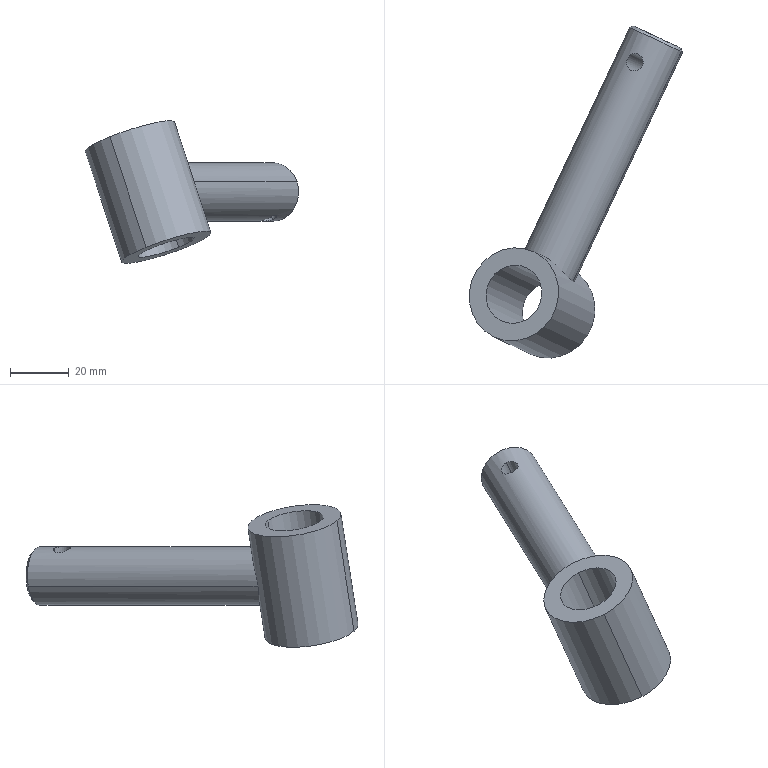Component | SolidWorks | FilmPressingSoilCoveringMechanism2Reverse-2_AttachedSoilWheelVerticalAxis2-1 | 1 solid | 13 faces | box 72.68 x 113.03 x 48.53 mm | volume 45663 mm3 | cylinder 8 | plane 3 | cone 2 | commonest cylinder face diameters 20 x4 6 x2 32 x2
build123d program:
from build123d import *

# Parameters (mm, degrees)
SKETCH1_R           = 16
BOSS_EXTRUDE1_DEPTH = 20
SKETCH2_R           = 10
BOSS_EXTRUDE2_DEPTH = 100
CHAMFER1_SIZE       = 1
SKETCH3_R           = 3
CUT_EXTRUDE1_DEPTH  = 50
SKETCH4_R           = 10
CUT_EXTRUDE2_DEPTH  = 109.885


with BuildPart() as part:
    # Sketch1 → Boss-Extrude1 (new, symmetric)
    with BuildSketch(Plane(origin=(0, 0, 0), x_dir=(1, 0, 0), z_dir=(0, 1, 0))):
        with Locations(Location((0, 0, 0), (0, 0, 270))):
            Circle(SKETCH1_R)
    extrude(amount=BOSS_EXTRUDE1_DEPTH, both=True)

    # Sketch2 → Boss-Extrude2 (add)
    with BuildSketch(Plane.XY):
        with Locations(Location((0, 0, 0), (0, 0, 180))):
            Circle(SKETCH2_R)
    extrude(amount=BOSS_EXTRUDE2_DEPTH)

    # Chamfer1
    chamfer1_edges = [part.edges().sort_by_distance(p)[0] for p in [
        (10, 0, 100),
    ]]
    chamfer(chamfer1_edges, length=CHAMFER1_SIZE)

    # Sketch3 → Cut-Extrude1 (cut, symmetric)
    with BuildSketch(Plane(origin=(0, 0, 0), x_dir=(1, 0, 0), z_dir=(0, 1, 0))):
        with Locations(Location((0, -89, 0), (0, 0, 270))):
            Circle(SKETCH3_R)
    extrude(amount=CUT_EXTRUDE1_DEPTH, both=True, mode=Mode.SUBTRACT)

    # Sketch4 → Cut-Extrude2 (cut, through all)
    with BuildSketch(Plane(origin=(0, 20, 0), x_dir=(1, 0, 0), z_dir=(0, 1, 0))):
        with Locations(Location((0, 0, 0), (0, 0, 270))):
            Circle(SKETCH4_R)
    extrude(amount=-CUT_EXTRUDE2_DEPTH, mode=Mode.SUBTRACT)


solid = part.part

# Placed as in the assembly
solid = solid.moved(Location((-1911.671, -307.604, 2567.971), (-90, 25.252, -20)))
STEP:
#1=COLOUR_RGB('',0.7922,0.8196,0.9333);
#2=FILL_AREA_STYLE_COLOUR('',#1);
#3=FILL_AREA_STYLE('',(#2));
#4=SURFACE_STYLE_FILL_AREA(#3);
#5=SURFACE_SIDE_STYLE('',(#4));
#6=SURFACE_STYLE_USAGE(.BOTH.,#5);
#7=PRESENTATION_STYLE_ASSIGNMENT((#6));
#8=CARTESIAN_POINT('',(-75.674,-12.352,101.841));
#9=VERTEX_POINT('',#8);
#10=CARTESIAN_POINT('',(-75.338,-11.639,101.841));
#11=VERTEX_POINT('',#10);
#12=CARTESIAN_POINT('',(-75.506,-11.995,101.841));
#13=DIRECTION('',(0.3093,-0.1459,-0.9397));
#14=DIRECTION('',(0.4266,0.9044,0.));
#15=AXIS2_PLACEMENT_3D('',#12,#13,#14);
#16=CIRCLE('',#15,0.3937);
#17=EDGE_CURVE('',#9,#11,#16,.T.);
#18=ORIENTED_EDGE('',*,*,#17,.F.);
#19=CARTESIAN_POINT('',(-75.187,-12.581,100.361));
#20=VERTEX_POINT('',#19);
#21=CARTESIAN_POINT('',(-75.674,-12.352,101.841));
#22=DIRECTION('',(0.3093,-0.1459,-0.9397));
#23=VECTOR('',#22,39.37);
#24=LINE('',#21,#23);
#25=EDGE_CURVE('',#9,#20,#24,.T.);
#26=ORIENTED_EDGE('',*,*,#25,.T.);
#27=CARTESIAN_POINT('',(-74.851,-11.869,100.361));
#28=VERTEX_POINT('',#27);
#29=CARTESIAN_POINT('',(-75.019,-12.225,100.361));
#30=DIRECTION('',(0.3093,-0.1459,-0.9397));
#31=DIRECTION('',(0.4266,0.9044,0.));
#32=AXIS2_PLACEMENT_3D('',#29,#30,#31);
#33=CIRCLE('',#32,0.3937);
#34=EDGE_CURVE('',#20,#28,#33,.T.);
#35=ORIENTED_EDGE('',*,*,#34,.T.);
#36=CARTESIAN_POINT('',(-75.338,-11.639,101.841));
#37=DIRECTION('',(0.3093,-0.1459,-0.9397));
#38=VECTOR('',#37,39.37);
#39=LINE('',#36,#38);
#40=EDGE_CURVE('',#11,#28,#39,.T.);
#41=ORIENTED_EDGE('',*,*,#40,.F.);
#42=EDGE_LOOP('',(#18,#26,#35,#41));
#43=FACE_OUTER_BOUND('',#42,.T.);
#44=CARTESIAN_POINT('',(-75.506,-11.995,101.841));
#45=DIRECTION('',(0.3093,-0.1459,-0.9397));
#46=DIRECTION('',(0.4266,0.9044,0.));
#47=AXIS2_PLACEMENT_3D('',#44,#45,#46);
#48=CYLINDRICAL_SURFACE('',#47,0.3937);
#49=ADVANCED_FACE('',(#43),#48,.F.);
#50=CARTESIAN_POINT('',(-73.94,-8.991,101.471));
#51=VERTEX_POINT('',#50);
#52=CARTESIAN_POINT('',(-73.839,-8.777,101.471));
#53=VERTEX_POINT('',#52);
#54=CARTESIAN_POINT('',(-73.94,-8.991,101.471));
#55=CARTESIAN_POINT('',(-73.947,-8.988,101.469));
#56=CARTESIAN_POINT('',(-73.953,-8.984,101.466));
#57=CARTESIAN_POINT('',(-73.964,-8.975,101.46));
#58=CARTESIAN_POINT('',(-73.969,-8.97,101.456));
#59=CARTESIAN_POINT('',(-73.978,-8.959,101.45));
#60=CARTESIAN_POINT('',(-73.982,-8.953,101.447));
#61=CARTESIAN_POINT('',(-73.989,-8.941,101.44));
#62=CARTESIAN_POINT('',(-73.992,-8.934,101.437));
#63=CARTESIAN_POINT('',(-73.995,-8.92,101.431));
#64=CARTESIAN_POINT('',(-73.997,-8.913,101.428));
#65=CARTESIAN_POINT('',(-73.998,-8.898,101.423));
#66=CARTESIAN_POINT('',(-73.998,-8.891,101.421));
#67=CARTESIAN_POINT('',(-73.996,-8.876,101.418));
#68=CARTESIAN_POINT('',(-73.995,-8.868,101.416));
#69=CARTESIAN_POINT('',(-73.99,-8.854,101.414));
#70=CARTESIAN_POINT('',(-73.988,-8.846,101.414));
#71=CARTESIAN_POINT('',(-73.981,-8.832,101.414));
#72=CARTESIAN_POINT('',(-73.977,-8.825,101.414));
#73=CARTESIAN_POINT('',(-73.968,-8.813,101.416));
#74=CARTESIAN_POINT('',(-73.964,-8.807,101.418));
#75=CARTESIAN_POINT('',(-73.948,-8.791,101.423));
#76=CARTESIAN_POINT('',(-73.935,-8.782,101.428));
#77=CARTESIAN_POINT('',(-73.916,-8.773,101.437));
#78=CARTESIAN_POINT('',(-73.909,-8.771,101.44));
#79=CARTESIAN_POINT('',(-73.895,-8.768,101.447));
#80=CARTESIAN_POINT('',(-73.888,-8.767,101.45));
#81=CARTESIAN_POINT('',(-73.874,-8.767,101.456));
#82=CARTESIAN_POINT('',(-73.867,-8.768,101.46));
#83=CARTESIAN_POINT('',(-73.853,-8.772,101.466));
#84=CARTESIAN_POINT('',(-73.846,-8.774,101.469));
#85=CARTESIAN_POINT('',(-73.839,-8.777,101.471));
#86=B_SPLINE_CURVE_WITH_KNOTS('',3,(#54,#55,#56,#57,#58,#59,#60,#61,#62,#63,#64,#65,#66,#67,#68,#69,#70,#71,#72,#73,#74,#75,#76,#77,#78,#79,#80,#81,#82,#83,#84,#85),.UNSPECIFIED.,.F.,.F.,(4,2,2,2,2,2,2,2,2,2,2,2,2,2,2,4),(0.009434,0.01002,0.01061,0.0112,0.01179,0.01238,0.01297,0.01356,0.01415,0.01474,0.01533,0.01651,0.0171,0.01769,0.01828,0.01887),.UNSPECIFIED.);
#87=EDGE_CURVE('',#51,#53,#86,.T.);
#88=ORIENTED_EDGE('',*,*,#87,.F.);
#89=CARTESIAN_POINT('',(-73.696,-9.106,100.731));
#90=VERTEX_POINT('',#89);
#91=CARTESIAN_POINT('',(-74.427,-8.761,102.951));
#92=DIRECTION('',(0.3093,-0.1459,-0.9397));
#93=VECTOR('',#92,39.37);
#94=LINE('',#91,#93);
#95=EDGE_CURVE('',#51,#90,#94,.T.);
#96=ORIENTED_EDGE('',*,*,#95,.T.);
#97=CARTESIAN_POINT('',(-73.596,-8.892,100.731));
#98=VERTEX_POINT('',#97);
#99=CARTESIAN_POINT('',(-73.596,-8.892,100.731));
#100=CARTESIAN_POINT('',(-73.602,-8.889,100.729));
#101=CARTESIAN_POINT('',(-73.609,-8.886,100.726));
#102=CARTESIAN_POINT('',(-73.624,-8.883,100.722));
#103=CARTESIAN_POINT('',(-73.631,-8.882,100.72));
#104=CARTESIAN_POINT('',(-73.647,-8.881,100.717));
#105=CARTESIAN_POINT('',(-73.654,-8.882,100.715));
#106=CARTESIAN_POINT('',(-73.669,-8.884,100.713));
#107=CARTESIAN_POINT('',(-73.677,-8.886,100.712));
#108=CARTESIAN_POINT('',(-73.699,-8.894,100.71));
#109=CARTESIAN_POINT('',(-73.713,-8.902,100.709));
#110=CARTESIAN_POINT('',(-73.73,-8.917,100.708));
#111=CARTESIAN_POINT('',(-73.735,-8.923,100.708));
#112=CARTESIAN_POINT('',(-73.745,-8.935,100.708));
#113=CARTESIAN_POINT('',(-73.749,-8.942,100.708));
#114=CARTESIAN_POINT('',(-73.755,-8.956,100.708));
#115=CARTESIAN_POINT('',(-73.758,-8.963,100.708));
#116=CARTESIAN_POINT('',(-73.762,-8.978,100.708));
#117=CARTESIAN_POINT('',(-73.763,-8.986,100.708));
#118=CARTESIAN_POINT('',(-73.763,-9.002,100.709));
#119=CARTESIAN_POINT('',(-73.763,-9.009,100.709));
#120=CARTESIAN_POINT('',(-73.76,-9.025,100.71));
#121=CARTESIAN_POINT('',(-73.758,-9.032,100.71));
#122=CARTESIAN_POINT('',(-73.753,-9.047,100.712));
#123=CARTESIAN_POINT('',(-73.749,-9.054,100.713));
#124=CARTESIAN_POINT('',(-73.742,-9.067,100.715));
#125=CARTESIAN_POINT('',(-73.737,-9.073,100.717));
#126=CARTESIAN_POINT('',(-73.727,-9.084,100.72));
#127=CARTESIAN_POINT('',(-73.721,-9.09,100.722));
#128=CARTESIAN_POINT('',(-73.709,-9.099,100.726));
#129=CARTESIAN_POINT('',(-73.703,-9.102,100.729));
#130=CARTESIAN_POINT('',(-73.696,-9.106,100.731));
#131=B_SPLINE_CURVE_WITH_KNOTS('',3,(#99,#100,#101,#102,#103,#104,#105,#106,#107,#108,#109,#110,#111,#112,#113,#114,#115,#116,#117,#118,#119,#120,#121,#122,#123,#124,#125,#126,#127,#128,#129,#130),.UNSPECIFIED.,.F.,.F.,(4,2,2,2,2,2,2,2,2,2,2,2,2,2,2,4),(0.,0.0005896,0.001179,0.001769,0.002359,0.003538,0.004127,0.004717,0.005307,0.005896,0.006486,0.007076,0.007665,0.008255,0.008844,0.009434),.UNSPECIFIED.);
#132=EDGE_CURVE('',#98,#90,#131,.T.);
#133=ORIENTED_EDGE('',*,*,#132,.F.);
#134=CARTESIAN_POINT('',(-74.326,-8.547,102.951));
#135=DIRECTION('',(0.3093,-0.1459,-0.9397));
#136=VECTOR('',#135,39.37);
#137=LINE('',#134,#136);
#138=EDGE_CURVE('',#53,#98,#137,.T.);
#139=ORIENTED_EDGE('',*,*,#138,.F.);
#140=EDGE_LOOP('',(#88,#96,#133,#139));
#141=FACE_OUTER_BOUND('',#140,.T.);
#142=CARTESIAN_POINT('',(-74.377,-8.654,102.951));
#143=DIRECTION('',(0.3093,-0.1459,-0.9397));
#144=DIRECTION('',(0.4266,0.9044,0.));
#145=AXIS2_PLACEMENT_3D('',#142,#143,#144);
#146=CYLINDRICAL_SURFACE('',#145,0.1181);
#147=ADVANCED_FACE('',(#141),#146,.F.);
#148=CARTESIAN_POINT('',(-73.282,-8.692,101.222));
#149=VERTEX_POINT('',#148);
#150=CARTESIAN_POINT('',(-73.884,-8.408,100.98));
#151=VERTEX_POINT('',#150);
#152=CARTESIAN_POINT('',(-73.583,-8.55,101.101));
#153=DIRECTION('',(0.4266,0.9044,0.));
#154=DIRECTION('',(0.8499,-0.4009,0.342));
#155=AXIS2_PLACEMENT_3D('',#152,#153,#154);
#156=CIRCLE('',#155,0.3543);
#157=EDGE_CURVE('',#149,#151,#156,.T.);
#158=ORIENTED_EDGE('',*,*,#157,.F.);
#159=CARTESIAN_POINT('',(-73.265,-8.743,101.236));
#160=VERTEX_POINT('',#159);
#161=CARTESIAN_POINT('',(-73.282,-8.692,101.222));
#162=DIRECTION('',(0.2993,-0.923,0.2418));
#163=VECTOR('',#162,39.37);
#164=LINE('',#161,#163);
#165=EDGE_CURVE('',#149,#160,#164,.T.);
#166=ORIENTED_EDGE('',*,*,#165,.T.);
#167=CARTESIAN_POINT('',(-73.935,-8.427,100.967));
#168=VERTEX_POINT('',#167);
#169=CARTESIAN_POINT('',(-73.6,-8.585,101.101));
#170=DIRECTION('',(-0.4266,-0.9044,-0.));
#171=DIRECTION('',(0.8499,-0.4009,0.342));
#172=AXIS2_PLACEMENT_3D('',#169,#170,#171);
#173=CIRCLE('',#172,0.3937);
#174=EDGE_CURVE('',#168,#160,#173,.T.);
#175=ORIENTED_EDGE('',*,*,#174,.F.);
#176=CARTESIAN_POINT('',(-73.884,-8.408,100.98));
#177=DIRECTION('',(-0.9026,-0.3561,-0.2418));
#178=VECTOR('',#177,39.37);
#179=LINE('',#176,#178);
#180=EDGE_CURVE('',#151,#168,#179,.T.);
#181=ORIENTED_EDGE('',*,*,#180,.F.);
#182=EDGE_LOOP('',(#158,#166,#175,#181));
#183=FACE_OUTER_BOUND('',#182,.T.);
#184=CARTESIAN_POINT('',(-73.583,-8.55,101.101));
#185=DIRECTION('',(-0.4266,-0.9044,-0.));
#186=DIRECTION('',(-0.8499,0.4009,-0.342));
#187=AXIS2_PLACEMENT_3D('',#184,#185,#186);
#188=CONICAL_SURFACE('',#187,0.3543,0.7854);
#189=ADVANCED_FACE('',(#183),#188,.T.);
#190=ORIENTED_EDGE('',*,*,#132,.T.);
#191=CARTESIAN_POINT('',(-73.696,-9.106,100.731));
#192=CARTESIAN_POINT('',(-73.69,-9.109,100.734));
#193=CARTESIAN_POINT('',(-73.683,-9.111,100.737));
#194=CARTESIAN_POINT('',(-73.669,-9.114,100.743));
#195=CARTESIAN_POINT('',(-73.662,-9.115,100.746));
#196=CARTESIAN_POINT('',(-73.648,-9.115,100.752));
#197=CARTESIAN_POINT('',(-73.641,-9.114,100.756));
#198=CARTESIAN_POINT('',(-73.627,-9.112,100.762));
#199=CARTESIAN_POINT('',(-73.62,-9.109,100.765));
#200=CARTESIAN_POINT('',(-73.607,-9.104,100.771));
#201=CARTESIAN_POINT('',(-73.601,-9.1,100.774));
#202=CARTESIAN_POINT('',(-73.589,-9.091,100.779));
#203=CARTESIAN_POINT('',(-73.583,-9.087,100.781));
#204=CARTESIAN_POINT('',(-73.572,-9.076,100.785));
#205=CARTESIAN_POINT('',(-73.567,-9.07,100.786));
#206=CARTESIAN_POINT('',(-73.559,-9.057,100.788));
#207=CARTESIAN_POINT('',(-73.555,-9.05,100.789));
#208=CARTESIAN_POINT('',(-73.548,-9.036,100.789));
#209=CARTESIAN_POINT('',(-73.545,-9.029,100.788));
#210=CARTESIAN_POINT('',(-73.541,-9.014,100.786));
#211=CARTESIAN_POINT('',(-73.54,-9.007,100.785));
#212=CARTESIAN_POINT('',(-73.537,-8.984,100.779));
#213=CARTESIAN_POINT('',(-73.538,-8.969,100.774));
#214=CARTESIAN_POINT('',(-73.544,-8.949,100.765));
#215=CARTESIAN_POINT('',(-73.547,-8.942,100.762));
#216=CARTESIAN_POINT('',(-73.553,-8.929,100.756));
#217=CARTESIAN_POINT('',(-73.557,-8.923,100.752));
#218=CARTESIAN_POINT('',(-73.566,-8.913,100.746));
#219=CARTESIAN_POINT('',(-73.572,-8.908,100.743));
#220=CARTESIAN_POINT('',(-73.583,-8.899,100.737));
#221=CARTESIAN_POINT('',(-73.589,-8.895,100.734));
#222=CARTESIAN_POINT('',(-73.596,-8.892,100.731));
#223=B_SPLINE_CURVE_WITH_KNOTS('',3,(#191,#192,#193,#194,#195,#196,#197,#198,#199,#200,#201,#202,#203,#204,#205,#206,#207,#208,#209,#210,#211,#212,#213,#214,#215,#216,#217,#218,#219,#220,#221,#222),.UNSPECIFIED.,.F.,.F.,(4,2,2,2,2,2,2,2,2,2,2,2,2,2,2,4),(0.009434,0.01002,0.01061,0.0112,0.01179,0.01238,0.01297,0.01356,0.01415,0.01474,0.01533,0.01651,0.0171,0.01769,0.01828,0.01887),.UNSPECIFIED.);
#224=EDGE_CURVE('',#90,#98,#223,.T.);
#225=ORIENTED_EDGE('',*,*,#224,.T.);
#226=EDGE_LOOP('',(#190,#225));
#227=FACE_BOUND('',#226,.T.);
#228=ORIENTED_EDGE('',*,*,#174,.T.);
#229=CARTESIAN_POINT('',(-74.718,-11.823,101.236));
#230=VERTEX_POINT('',#229);
#231=CARTESIAN_POINT('',(-73.249,-8.707,101.236));
#232=DIRECTION('',(-0.4266,-0.9044,-0.));
#233=VECTOR('',#232,39.37);
#234=LINE('',#231,#233);
#235=EDGE_CURVE('',#160,#230,#234,.T.);
#236=ORIENTED_EDGE('',*,*,#235,.T.);
#237=CARTESIAN_POINT('',(-74.872,-11.598,100.731));
#238=VERTEX_POINT('',#237);
#239=CARTESIAN_POINT('',(-74.718,-11.823,101.236));
#240=CARTESIAN_POINT('',(-74.71,-11.827,101.211));
#241=CARTESIAN_POINT('',(-74.703,-11.828,101.185));
#242=CARTESIAN_POINT('',(-74.695,-11.825,101.146));
#243=CARTESIAN_POINT('',(-74.693,-11.823,101.133));
#244=CARTESIAN_POINT('',(-74.69,-11.819,101.107));
#245=CARTESIAN_POINT('',(-74.688,-11.816,101.094));
#246=CARTESIAN_POINT('',(-74.685,-11.805,101.056));
#247=CARTESIAN_POINT('',(-74.685,-11.796,101.031));
#248=CARTESIAN_POINT('',(-74.689,-11.776,100.982));
#249=CARTESIAN_POINT('',(-74.693,-11.764,100.958));
#250=CARTESIAN_POINT('',(-74.702,-11.746,100.924));
#251=CARTESIAN_POINT('',(-74.705,-11.739,100.913));
#252=CARTESIAN_POINT('',(-74.713,-11.726,100.891));
#253=CARTESIAN_POINT('',(-74.718,-11.719,100.88));
#254=CARTESIAN_POINT('',(-74.733,-11.699,100.85));
#255=CARTESIAN_POINT('',(-74.745,-11.686,100.831));
#256=CARTESIAN_POINT('',(-74.774,-11.659,100.795));
#257=CARTESIAN_POINT('',(-74.791,-11.645,100.779));
#258=CARTESIAN_POINT('',(-74.819,-11.627,100.759));
#259=CARTESIAN_POINT('',(-74.829,-11.621,100.753));
#260=CARTESIAN_POINT('',(-74.85,-11.609,100.741));
#261=CARTESIAN_POINT('',(-74.861,-11.603,100.736));
#262=CARTESIAN_POINT('',(-74.872,-11.598,100.731));
#263=B_SPLINE_CURVE_WITH_KNOTS('',3,(#239,#240,#241,#242,#243,#244,#245,#246,#247,#248,#249,#250,#251,#252,#253,#254,#255,#256,#257,#258,#259,#260,#261,#262),.UNSPECIFIED.,.F.,.F.,(4,2,2,2,2,2,2,2,2,2,2,4),(0.03215,0.03416,0.03516,0.03616,0.03817,0.04017,0.04118,0.04218,0.04419,0.04619,0.0472,0.0482),.UNSPECIFIED.);
#264=EDGE_CURVE('',#230,#238,#263,.T.);
#265=ORIENTED_EDGE('',*,*,#264,.T.);
#266=CARTESIAN_POINT('',(-75.387,-11.508,100.967));
#267=VERTEX_POINT('',#266);
#268=CARTESIAN_POINT('',(-74.872,-11.598,100.731));
#269=CARTESIAN_POINT('',(-74.895,-11.587,100.722));
#270=CARTESIAN_POINT('',(-74.919,-11.578,100.716));
#271=CARTESIAN_POINT('',(-74.956,-11.566,100.71));
#272=CARTESIAN_POINT('',(-74.969,-11.562,100.709));
#273=CARTESIAN_POINT('',(-74.994,-11.555,100.707));
#274=CARTESIAN_POINT('',(-75.007,-11.552,100.707));
#275=CARTESIAN_POINT('',(-75.033,-11.546,100.709));
#276=CARTESIAN_POINT('',(-75.046,-11.544,100.71));
#277=CARTESIAN_POINT('',(-75.072,-11.539,100.714));
#278=CARTESIAN_POINT('',(-75.085,-11.538,100.716));
#279=CARTESIAN_POINT('',(-75.123,-11.532,100.726));
#280=CARTESIAN_POINT('',(-75.148,-11.53,100.734));
#281=CARTESIAN_POINT('',(-75.185,-11.527,100.75));
#282=CARTESIAN_POINT('',(-75.197,-11.527,100.756));
#283=CARTESIAN_POINT('',(-75.22,-11.525,100.769));
#284=CARTESIAN_POINT('',(-75.231,-11.525,100.776));
#285=CARTESIAN_POINT('',(-75.264,-11.523,100.798));
#286=CARTESIAN_POINT('',(-75.285,-11.523,100.814));
#287=CARTESIAN_POINT('',(-75.313,-11.521,100.843));
#288=CARTESIAN_POINT('',(-75.322,-11.52,100.852));
#289=CARTESIAN_POINT('',(-75.339,-11.519,100.873));
#290=CARTESIAN_POINT('',(-75.346,-11.518,100.884));
#291=CARTESIAN_POINT('',(-75.36,-11.516,100.906));
#292=CARTESIAN_POINT('',(-75.367,-11.515,100.918));
#293=CARTESIAN_POINT('',(-75.378,-11.511,100.942));
#294=CARTESIAN_POINT('',(-75.383,-11.51,100.954));
#295=CARTESIAN_POINT('',(-75.387,-11.508,100.967));
#296=B_SPLINE_CURVE_WITH_KNOTS('',3,(#268,#269,#270,#271,#272,#273,#274,#275,#276,#277,#278,#279,#280,#281,#282,#283,#284,#285,#286,#287,#288,#289,#290,#291,#292,#293,#294,#295),.UNSPECIFIED.,.F.,.F.,(4,2,2,2,2,2,2,2,2,2,2,2,2,4),(0.0482,0.0502,0.0512,0.0522,0.0532,0.0542,0.05621,0.05721,0.05821,0.06021,0.06121,0.06221,0.06321,0.06421),.UNSPECIFIED.);
#297=EDGE_CURVE('',#238,#267,#296,.T.);
#298=ORIENTED_EDGE('',*,*,#297,.T.);
#299=CARTESIAN_POINT('',(-73.918,-8.392,100.967));
#300=DIRECTION('',(-0.4266,-0.9044,-0.));
#301=VECTOR('',#300,39.37);
#302=LINE('',#299,#301);
#303=EDGE_CURVE('',#168,#267,#302,.T.);
#304=ORIENTED_EDGE('',*,*,#303,.F.);
#305=EDGE_LOOP('',(#228,#236,#265,#298,#304));
#306=FACE_OUTER_BOUND('',#305,.T.);
#307=CARTESIAN_POINT('',(-73.583,-8.55,101.101));
#308=DIRECTION('',(-0.4266,-0.9044,-0.));
#309=DIRECTION('',(-0.8499,0.4009,-0.342));
#310=AXIS2_PLACEMENT_3D('',#307,#308,#309);
#311=CYLINDRICAL_SURFACE('',#310,0.3937);
#312=ADVANCED_FACE('',(#227,#306),#311,.T.);
#313=CARTESIAN_POINT('',(-74.75,-11.656,100.361));
#314=VERTEX_POINT('',#313);
#315=CARTESIAN_POINT('',(-75.288,-12.795,100.361));
#316=VERTEX_POINT('',#315);
#317=CARTESIAN_POINT('',(-75.019,-12.225,100.361));
#318=DIRECTION('',(0.3093,-0.1459,-0.9397));
#319=DIRECTION('',(0.4266,0.9044,0.));
#320=AXIS2_PLACEMENT_3D('',#317,#318,#319);
#321=CIRCLE('',#320,0.6299);
#322=EDGE_CURVE('',#314,#316,#321,.T.);
#323=ORIENTED_EDGE('',*,*,#322,.F.);
#324=CARTESIAN_POINT('',(-74.75,-11.656,100.361));
#325=DIRECTION('',(-0.3093,0.1459,0.9397));
#326=VECTOR('',#325,39.37);
#327=LINE('',#324,#326);
#328=EDGE_CURVE('',#314,#238,#327,.T.);
#329=ORIENTED_EDGE('',*,*,#328,.T.);
#330=ORIENTED_EDGE('',*,*,#264,.F.);
#331=CARTESIAN_POINT('',(-75.116,-11.483,101.471));
#332=VERTEX_POINT('',#331);
#333=CARTESIAN_POINT('',(-75.116,-11.483,101.471));
#334=CARTESIAN_POINT('',(-75.104,-11.489,101.476));
#335=CARTESIAN_POINT('',(-75.093,-11.494,101.48));
#336=CARTESIAN_POINT('',(-75.07,-11.507,101.486));
#337=CARTESIAN_POINT('',(-75.059,-11.513,101.489));
#338=CARTESIAN_POINT('',(-75.037,-11.527,101.493));
#339=CARTESIAN_POINT('',(-75.026,-11.535,101.494));
#340=CARTESIAN_POINT('',(-75.005,-11.55,101.495));
#341=CARTESIAN_POINT('',(-74.994,-11.558,101.495));
#342=CARTESIAN_POINT('',(-74.963,-11.583,101.493));
#343=CARTESIAN_POINT('',(-74.943,-11.6,101.489));
#344=CARTESIAN_POINT('',(-74.905,-11.636,101.477));
#345=CARTESIAN_POINT('',(-74.887,-11.653,101.468));
#346=CARTESIAN_POINT('',(-74.862,-11.68,101.452));
#347=CARTESIAN_POINT('',(-74.854,-11.688,101.446));
#348=CARTESIAN_POINT('',(-74.838,-11.706,101.434));
#349=CARTESIAN_POINT('',(-74.83,-11.714,101.427));
#350=CARTESIAN_POINT('',(-74.808,-11.739,101.404));
#351=CARTESIAN_POINT('',(-74.795,-11.754,101.388));
#352=CARTESIAN_POINT('',(-74.776,-11.774,101.36));
#353=CARTESIAN_POINT('',(-74.77,-11.781,101.35));
#354=CARTESIAN_POINT('',(-74.758,-11.793,101.329));
#355=CARTESIAN_POINT('',(-74.752,-11.798,101.318));
#356=CARTESIAN_POINT('',(-74.741,-11.808,101.296));
#357=CARTESIAN_POINT('',(-74.736,-11.812,101.285));
#358=CARTESIAN_POINT('',(-74.727,-11.819,101.261));
#359=CARTESIAN_POINT('',(-74.722,-11.822,101.248));
#360=CARTESIAN_POINT('',(-74.718,-11.823,101.236));
#361=B_SPLINE_CURVE_WITH_KNOTS('',3,(#333,#334,#335,#336,#337,#338,#339,#340,#341,#342,#343,#344,#345,#346,#347,#348,#349,#350,#351,#352,#353,#354,#355,#356,#357,#358,#359,#360),.UNSPECIFIED.,.F.,.F.,(4,2,2,2,2,2,2,2,2,2,2,2,2,4),(0.0161,0.0171,0.0181,0.01911,0.02011,0.02212,0.02412,0.02513,0.02613,0.02814,0.02914,0.03014,0.03115,0.03215),.UNSPECIFIED.);
#362=EDGE_CURVE('',#332,#230,#361,.T.);
#363=ORIENTED_EDGE('',*,*,#362,.F.);
#364=CARTESIAN_POINT('',(-75.237,-11.426,101.841));
#365=VERTEX_POINT('',#364);
#366=CARTESIAN_POINT('',(-74.75,-11.656,100.361));
#367=DIRECTION('',(-0.3093,0.1459,0.9397));
#368=VECTOR('',#367,39.37);
#369=LINE('',#366,#368);
#370=EDGE_CURVE('',#332,#365,#369,.T.);
#371=ORIENTED_EDGE('',*,*,#370,.T.);
#372=CARTESIAN_POINT('',(-75.775,-12.565,101.841));
#373=VERTEX_POINT('',#372);
#374=CARTESIAN_POINT('',(-75.506,-11.995,101.841));
#375=DIRECTION('',(0.3093,-0.1459,-0.9397));
#376=DIRECTION('',(0.4266,0.9044,0.));
#377=AXIS2_PLACEMENT_3D('',#374,#375,#376);
#378=CIRCLE('',#377,0.6299);
#379=EDGE_CURVE('',#365,#373,#378,.T.);
#380=ORIENTED_EDGE('',*,*,#379,.T.);
#381=CARTESIAN_POINT('',(-75.288,-12.795,100.361));
#382=DIRECTION('',(-0.3093,0.1459,0.9397));
#383=VECTOR('',#382,39.37);
#384=LINE('',#381,#383);
#385=EDGE_CURVE('',#316,#373,#384,.T.);
#386=ORIENTED_EDGE('',*,*,#385,.F.);
#387=EDGE_LOOP('',(#323,#329,#330,#363,#371,#380,#386));
#388=FACE_OUTER_BOUND('',#387,.T.);
#389=CARTESIAN_POINT('',(-75.019,-12.225,100.361));
#390=DIRECTION('',(-0.3093,0.1459,0.9397));
#391=DIRECTION('',(-0.4266,-0.9044,-0.));
#392=AXIS2_PLACEMENT_3D('',#389,#390,#391);
#393=CYLINDRICAL_SURFACE('',#392,0.6299);
#394=ADVANCED_FACE('',(#388),#393,.T.);
#395=ORIENTED_EDGE('',*,*,#328,.F.);
#396=CARTESIAN_POINT('',(-75.019,-12.225,100.361));
#397=DIRECTION('',(0.3093,-0.1459,-0.9397));
#398=DIRECTION('',(0.4266,0.9044,0.));
#399=AXIS2_PLACEMENT_3D('',#396,#397,#398);
#400=CIRCLE('',#399,0.6299);
#401=EDGE_CURVE('',#316,#314,#400,.T.);
#402=ORIENTED_EDGE('',*,*,#401,.F.);
#403=ORIENTED_EDGE('',*,*,#385,.T.);
#404=CARTESIAN_POINT('',(-75.506,-11.995,101.841));
#405=DIRECTION('',(0.3093,-0.1459,-0.9397));
#406=DIRECTION('',(0.4266,0.9044,0.));
#407=AXIS2_PLACEMENT_3D('',#404,#405,#406);
#408=CIRCLE('',#407,0.6299);
#409=EDGE_CURVE('',#373,#365,#408,.T.);
#410=ORIENTED_EDGE('',*,*,#409,.T.);
#411=ORIENTED_EDGE('',*,*,#370,.F.);
#412=CARTESIAN_POINT('',(-75.387,-11.508,100.967));
#413=CARTESIAN_POINT('',(-75.396,-11.504,100.992));
#414=CARTESIAN_POINT('',(-75.401,-11.499,101.017));
#415=CARTESIAN_POINT('',(-75.403,-11.491,101.056));
#416=CARTESIAN_POINT('',(-75.403,-11.488,101.069));
#417=CARTESIAN_POINT('',(-75.402,-11.483,101.095));
#418=CARTESIAN_POINT('',(-75.401,-11.48,101.108));
#419=CARTESIAN_POINT('',(-75.394,-11.471,101.147));
#420=CARTESIAN_POINT('',(-75.388,-11.465,101.172));
#421=CARTESIAN_POINT('',(-75.369,-11.455,101.221));
#422=CARTESIAN_POINT('',(-75.358,-11.451,101.244));
#423=CARTESIAN_POINT('',(-75.338,-11.445,101.278));
#424=CARTESIAN_POINT('',(-75.331,-11.444,101.29));
#425=CARTESIAN_POINT('',(-75.316,-11.442,101.311));
#426=CARTESIAN_POINT('',(-75.308,-11.441,101.322));
#427=CARTESIAN_POINT('',(-75.282,-11.44,101.353));
#428=CARTESIAN_POINT('',(-75.264,-11.441,101.372));
#429=CARTESIAN_POINT('',(-75.235,-11.445,101.398));
#430=CARTESIAN_POINT('',(-75.225,-11.447,101.407));
#431=CARTESIAN_POINT('',(-75.204,-11.451,101.423));
#432=CARTESIAN_POINT('',(-75.193,-11.454,101.43));
#433=CARTESIAN_POINT('',(-75.161,-11.464,101.451));
#434=CARTESIAN_POINT('',(-75.138,-11.473,101.462));
#435=CARTESIAN_POINT('',(-75.116,-11.483,101.471));
#436=B_SPLINE_CURVE_WITH_KNOTS('',3,(#412,#413,#414,#415,#416,#417,#418,#419,#420,#421,#422,#423,#424,#425,#426,#427,#428,#429,#430,#431,#432,#433,#434,#435),.UNSPECIFIED.,.F.,.F.,(4,2,2,2,2,2,2,2,2,2,2,4),(0.,0.002012,0.003018,0.004024,0.006036,0.008048,0.009054,0.01006,0.01207,0.01308,0.01408,0.0161),.UNSPECIFIED.);
#437=EDGE_CURVE('',#267,#332,#436,.T.);
#438=ORIENTED_EDGE('',*,*,#437,.F.);
#439=ORIENTED_EDGE('',*,*,#297,.F.);
#440=EDGE_LOOP('',(#395,#402,#403,#410,#411,#438,#439));
#441=FACE_OUTER_BOUND('',#440,.T.);
#442=CARTESIAN_POINT('',(-75.019,-12.225,100.361));
#443=DIRECTION('',(-0.3093,0.1459,0.9397));
#444=DIRECTION('',(-0.4266,-0.9044,-0.));
#445=AXIS2_PLACEMENT_3D('',#442,#443,#444);
#446=CYLINDRICAL_SURFACE('',#445,0.6299);
#447=ADVANCED_FACE('',(#441),#446,.T.);
#448=CARTESIAN_POINT('',(-75.019,-12.225,100.361));
#449=DIRECTION('',(0.3093,-0.1459,-0.9397));
#450=DIRECTION('',(0.4266,0.9044,0.));
#451=AXIS2_PLACEMENT_3D('',#448,#449,#450);
#452=CIRCLE('',#451,0.3937);
#453=EDGE_CURVE('',#28,#20,#452,.T.);
#454=ORIENTED_EDGE('',*,*,#453,.F.);
#455=ORIENTED_EDGE('',*,*,#34,.F.);
#456=EDGE_LOOP('',(#454,#455));
#457=FACE_BOUND('',#456,.T.);
#458=ORIENTED_EDGE('',*,*,#401,.T.);
#459=ORIENTED_EDGE('',*,*,#322,.T.);
#460=EDGE_LOOP('',(#458,#459));
#461=FACE_OUTER_BOUND('',#460,.T.);
#462=CARTESIAN_POINT('',(-75.019,-12.225,100.361));
#463=DIRECTION('',(0.3093,-0.1459,-0.9397));
#464=DIRECTION('',(0.4266,0.9044,0.));
#465=AXIS2_PLACEMENT_3D('',#462,#463,#464);
#466=PLANE('',#465);
#467=ADVANCED_FACE('',(#457,#461),#466,.T.);
#468=CARTESIAN_POINT('',(-75.506,-11.995,101.841));
#469=DIRECTION('',(0.3093,-0.1459,-0.9397));
#470=DIRECTION('',(0.4266,0.9044,0.));
#471=AXIS2_PLACEMENT_3D('',#468,#469,#470);
#472=CIRCLE('',#471,0.3937);
#473=EDGE_CURVE('',#11,#9,#472,.T.);
#474=ORIENTED_EDGE('',*,*,#473,.T.);
#475=ORIENTED_EDGE('',*,*,#17,.T.);
#476=EDGE_LOOP('',(#474,#475));
#477=FACE_BOUND('',#476,.T.);
#478=ORIENTED_EDGE('',*,*,#409,.F.);
#479=ORIENTED_EDGE('',*,*,#379,.F.);
#480=EDGE_LOOP('',(#478,#479));
#481=FACE_OUTER_BOUND('',#480,.T.);
#482=CARTESIAN_POINT('',(-75.506,-11.995,101.841));
#483=DIRECTION('',(0.3093,-0.1459,-0.9397));
#484=DIRECTION('',(0.4266,0.9044,0.));
#485=AXIS2_PLACEMENT_3D('',#482,#483,#484);
#486=PLANE('',#485);
#487=ADVANCED_FACE('',(#477,#481),#486,.F.);
#488=ORIENTED_EDGE('',*,*,#235,.F.);
#489=CARTESIAN_POINT('',(-73.6,-8.585,101.101));
#490=DIRECTION('',(-0.4266,-0.9044,-0.));
#491=DIRECTION('',(0.8499,-0.4009,0.342));
#492=AXIS2_PLACEMENT_3D('',#489,#490,#491);
#493=CIRCLE('',#492,0.3937);
#494=EDGE_CURVE('',#160,#168,#493,.T.);
#495=ORIENTED_EDGE('',*,*,#494,.T.);
#496=ORIENTED_EDGE('',*,*,#303,.T.);
#497=ORIENTED_EDGE('',*,*,#437,.T.);
#498=ORIENTED_EDGE('',*,*,#362,.T.);
#499=EDGE_LOOP('',(#488,#495,#496,#497,#498));
#500=FACE_OUTER_BOUND('',#499,.T.);
#501=CARTESIAN_POINT('',(-73.839,-8.777,101.471));
#502=CARTESIAN_POINT('',(-73.833,-8.78,101.474));
#503=CARTESIAN_POINT('',(-73.826,-8.784,101.476));
#504=CARTESIAN_POINT('',(-73.814,-8.793,101.481));
#505=CARTESIAN_POINT('',(-73.809,-8.798,101.483));
#506=CARTESIAN_POINT('',(-73.799,-8.809,101.486));
#507=CARTESIAN_POINT('',(-73.794,-8.816,101.487));
#508=CARTESIAN_POINT('',(-73.786,-8.829,101.49));
#509=CARTESIAN_POINT('',(-73.783,-8.836,101.491));
#510=CARTESIAN_POINT('',(-73.775,-8.858,101.493));
#511=CARTESIAN_POINT('',(-73.772,-8.873,101.494));
#512=CARTESIAN_POINT('',(-73.773,-8.896,101.494));
#513=CARTESIAN_POINT('',(-73.774,-8.904,101.494));
#514=CARTESIAN_POINT('',(-73.778,-8.919,101.495));
#515=CARTESIAN_POINT('',(-73.78,-8.927,101.495));
#516=CARTESIAN_POINT('',(-73.787,-8.941,101.495));
#517=CARTESIAN_POINT('',(-73.791,-8.948,101.495));
#518=CARTESIAN_POINT('',(-73.8,-8.96,101.494));
#519=CARTESIAN_POINT('',(-73.806,-8.966,101.494));
#520=CARTESIAN_POINT('',(-73.817,-8.976,101.494));
#521=CARTESIAN_POINT('',(-73.824,-8.981,101.493));
#522=CARTESIAN_POINT('',(-73.837,-8.988,101.493));
#523=CARTESIAN_POINT('',(-73.844,-8.992,101.492));
#524=CARTESIAN_POINT('',(-73.859,-8.997,101.491));
#525=CARTESIAN_POINT('',(-73.866,-8.999,101.49));
#526=CARTESIAN_POINT('',(-73.882,-9.001,101.487));
#527=CARTESIAN_POINT('',(-73.889,-9.001,101.486));
#528=CARTESIAN_POINT('',(-73.904,-9.001,101.483));
#529=CARTESIAN_POINT('',(-73.912,-9.,101.481));
#530=CARTESIAN_POINT('',(-73.926,-8.996,101.476));
#531=CARTESIAN_POINT('',(-73.933,-8.994,101.474));
#532=CARTESIAN_POINT('',(-73.94,-8.991,101.471));
#533=B_SPLINE_CURVE_WITH_KNOTS('',3,(#501,#502,#503,#504,#505,#506,#507,#508,#509,#510,#511,#512,#513,#514,#515,#516,#517,#518,#519,#520,#521,#522,#523,#524,#525,#526,#527,#528,#529,#530,#531,#532),.UNSPECIFIED.,.F.,.F.,(4,2,2,2,2,2,2,2,2,2,2,2,2,2,2,4),(0.,0.0005896,0.001179,0.001769,0.002359,0.003538,0.004127,0.004717,0.005307,0.005896,0.006486,0.007076,0.007665,0.008255,0.008844,0.009434),.UNSPECIFIED.);
#534=EDGE_CURVE('',#53,#51,#533,.T.);
#535=ORIENTED_EDGE('',*,*,#534,.T.);
#536=ORIENTED_EDGE('',*,*,#87,.T.);
#537=EDGE_LOOP('',(#535,#536));
#538=FACE_BOUND('',#537,.T.);
#539=CARTESIAN_POINT('',(-73.583,-8.55,101.101));
#540=DIRECTION('',(-0.4266,-0.9044,-0.));
#541=DIRECTION('',(-0.8499,0.4009,-0.342));
#542=AXIS2_PLACEMENT_3D('',#539,#540,#541);
#543=CYLINDRICAL_SURFACE('',#542,0.3937);
#544=ADVANCED_FACE('',(#500,#538),#543,.T.);
#545=CARTESIAN_POINT('',(-73.583,-8.55,101.101));
#546=DIRECTION('',(0.4266,0.9044,0.));
#547=DIRECTION('',(0.8499,-0.4009,0.342));
#548=AXIS2_PLACEMENT_3D('',#545,#546,#547);
#549=CIRCLE('',#548,0.3543);
#550=EDGE_CURVE('',#151,#149,#549,.T.);
#551=ORIENTED_EDGE('',*,*,#550,.T.);
#552=ORIENTED_EDGE('',*,*,#157,.T.);
#553=EDGE_LOOP('',(#551,#552));
#554=FACE_OUTER_BOUND('',#553,.T.);
#555=CARTESIAN_POINT('',(-73.583,-8.55,101.101));
#556=DIRECTION('',(0.4266,0.9044,0.));
#557=DIRECTION('',(0.8499,-0.4009,0.342));
#558=AXIS2_PLACEMENT_3D('',#555,#556,#557);
#559=PLANE('',#558);
#560=ADVANCED_FACE('',(#554),#559,.T.);
#561=ORIENTED_EDGE('',*,*,#165,.F.);
#562=ORIENTED_EDGE('',*,*,#550,.F.);
#563=ORIENTED_EDGE('',*,*,#180,.T.);
#564=ORIENTED_EDGE('',*,*,#494,.F.);
#565=EDGE_LOOP('',(#561,#562,#563,#564));
#566=FACE_OUTER_BOUND('',#565,.T.);
#567=CARTESIAN_POINT('',(-73.583,-8.55,101.101));
#568=DIRECTION('',(-0.4266,-0.9044,-0.));
#569=DIRECTION('',(-0.8499,0.4009,-0.342));
#570=AXIS2_PLACEMENT_3D('',#567,#568,#569);
#571=CONICAL_SURFACE('',#570,0.3543,0.7854);
#572=ADVANCED_FACE('',(#566),#571,.T.);
#573=ORIENTED_EDGE('',*,*,#95,.F.);
#574=ORIENTED_EDGE('',*,*,#534,.F.);
#575=ORIENTED_EDGE('',*,*,#138,.T.);
#576=ORIENTED_EDGE('',*,*,#224,.F.);
#577=EDGE_LOOP('',(#573,#574,#575,#576));
#578=FACE_OUTER_BOUND('',#577,.T.);
#579=CARTESIAN_POINT('',(-74.377,-8.654,102.951));
#580=DIRECTION('',(0.3093,-0.1459,-0.9397));
#581=DIRECTION('',(0.4266,0.9044,0.));
#582=AXIS2_PLACEMENT_3D('',#579,#580,#581);
#583=CYLINDRICAL_SURFACE('',#582,0.1181);
#584=ADVANCED_FACE('',(#578),#583,.F.);
#585=ORIENTED_EDGE('',*,*,#25,.F.);
#586=ORIENTED_EDGE('',*,*,#473,.F.);
#587=ORIENTED_EDGE('',*,*,#40,.T.);
#588=ORIENTED_EDGE('',*,*,#453,.T.);
#589=EDGE_LOOP('',(#585,#586,#587,#588));
#590=FACE_OUTER_BOUND('',#589,.T.);
#591=CARTESIAN_POINT('',(-75.506,-11.995,101.841));
#592=DIRECTION('',(0.3093,-0.1459,-0.9397));
#593=DIRECTION('',(0.4266,0.9044,0.));
#594=AXIS2_PLACEMENT_3D('',#591,#592,#593);
#595=CYLINDRICAL_SURFACE('',#594,0.3937);
#596=ADVANCED_FACE('',(#590),#595,.F.);
#597=CLOSED_SHELL('',(#49,#147,#189,#312,#394,#447,#467,#487,#544,#560,#572,#584,#596));
#598=MANIFOLD_SOLID_BREP('',#597);
#599=STYLED_ITEM('',(#7),#598);
#600=(LENGTH_UNIT()NAMED_UNIT(*)SI_UNIT($,.METRE.));
#601=LENGTH_MEASURE_WITH_UNIT(LENGTH_MEASURE(0.0254),#600);
#602=DIMENSIONAL_EXPONENTS(1.,0.,0.,0.,0.,0.,0.);
#603=(CONVERSION_BASED_UNIT('',#601)LENGTH_UNIT()NAMED_UNIT(#602));
#604=UNCERTAINTY_MEASURE_WITH_UNIT(LENGTH_MEASURE(0.00001),#603,'','');
#605=(NAMED_UNIT(*)PLANE_ANGLE_UNIT()SI_UNIT($,.RADIAN.));
#606=(NAMED_UNIT(*)SI_UNIT($,.STERADIAN.)SOLID_ANGLE_UNIT());
#607=(GEOMETRIC_REPRESENTATION_CONTEXT(3)GLOBAL_UNCERTAINTY_ASSIGNED_CONTEXT((#604))GLOBAL_UNIT_ASSIGNED_CONTEXT((#603,#605,#606))REPRESENTATION_CONTEXT('',''));
#608=MECHANICAL_DESIGN_GEOMETRIC_PRESENTATION_REPRESENTATION('',(#599),#607);
#609=CARTESIAN_POINT('',(0.,0.,0.));
#610=DIRECTION('',(0.,0.,1.));
#611=DIRECTION('',(1.,0.,0.));
#612=AXIS2_PLACEMENT_3D('',#609,#610,#611);
#613=(LENGTH_UNIT()NAMED_UNIT(*)SI_UNIT($,.METRE.));
#614=LENGTH_MEASURE_WITH_UNIT(LENGTH_MEASURE(0.0254),#613);
#615=DIMENSIONAL_EXPONENTS(1.,0.,0.,0.,0.,0.,0.);
#616=(CONVERSION_BASED_UNIT('',#614)LENGTH_UNIT()NAMED_UNIT(#615));
#617=UNCERTAINTY_MEASURE_WITH_UNIT(LENGTH_MEASURE(0.00001),#616,'','');
#618=(NAMED_UNIT(*)PLANE_ANGLE_UNIT()SI_UNIT($,.RADIAN.));
#619=(NAMED_UNIT(*)SI_UNIT($,.STERADIAN.)SOLID_ANGLE_UNIT());
#620=(GEOMETRIC_REPRESENTATION_CONTEXT(3)GLOBAL_UNCERTAINTY_ASSIGNED_CONTEXT((#617))GLOBAL_UNIT_ASSIGNED_CONTEXT((#616,#618,#619))REPRESENTATION_CONTEXT('',''));
#621=ADVANCED_BREP_SHAPE_REPRESENTATION('',(#598,#612),#620);
#622=PRESENTATION_LAYER_ASSIGNMENT('','',(#599));